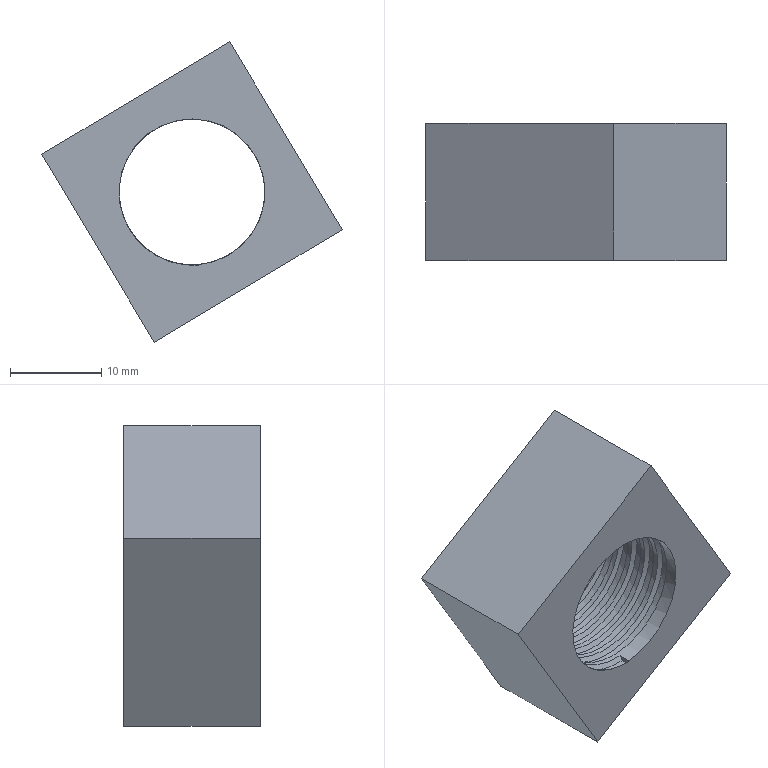Component | NX | SQUARE_NUT | 1 solid | 11 faces | volume 5414 mm3 | plane 7 | cylinder 2 | spline 2 | commonest cylinder face diameters 16 x1 17 x1